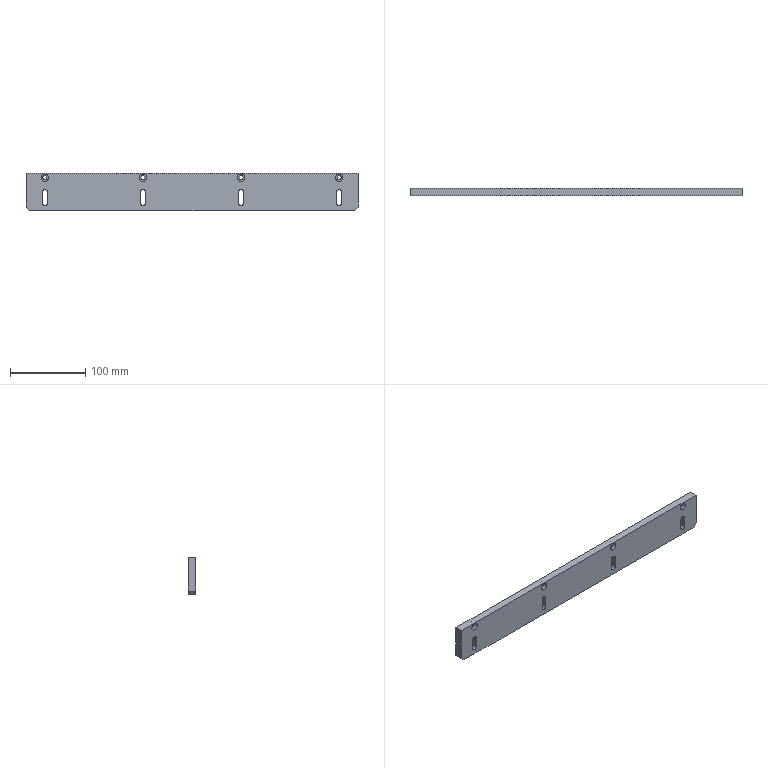Component | SolidWorks | 002MaterialPickingModuleB-1_J-019-1 | 1 solid | 48 faces | box 440 x 10 x 50 mm | volume 212389 mm3 | cylinder 28 | plane 20 | commonest cylinder face diameters 6.5 x12 10 x8 5.5 x8 | material 45
build123d program:
from build123d import *

# Parameters (mm, degrees)
SKETCH1_W                                       = 440
SKETCH1_H                                       = 50
BOSS_EXTRUDE1_DEPTH                             = 10
CHAMFER1_SIZE                                   = 5
M5_HEX_SOCKET_HEAD_CAP_SCREW_CBORE1_D           = 5.5
M5_HEX_SOCKET_HEAD_CAP_SCREW_CBORE1_CBORE_D     = 10
M5_HEX_SOCKET_HEAD_CAP_SCREW_CBORE1_CBORE_DEPTH = 5.4
CUT_EXTRUDE1_DEPTH                              = 222.642


with BuildPart() as part:
    # Sketch1 → Boss-Extrude1 (new body)
    with BuildSketch(Plane(origin=(0, 0, 0), x_dir=(1, 0, 0), z_dir=(0, 1, 0))):
        Rectangle(SKETCH1_W, SKETCH1_H)
    extrude(amount=BOSS_EXTRUDE1_DEPTH)

    # Chamfer1
    chamfer1_edges = [part.edges().sort_by_distance(p)[0] for p in [
        (-220, 5, -25),
        (220, 5, -25),
    ]]
    chamfer(chamfer1_edges, length=CHAMFER1_SIZE)

    # M5 Hex Socket Head Cap Screw CBORE1 (through all)
    with Locations(Plane(origin=(0, 0, 0), x_dir=(-1, 0, 0), z_dir=(0, -1, 0))):
        with Locations((-195, -19), (-65, -19), (65, -19), (195, -19)):
            CounterBoreHole(M5_HEX_SOCKET_HEAD_CAP_SCREW_CBORE1_D / 2, M5_HEX_SOCKET_HEAD_CAP_SCREW_CBORE1_CBORE_D / 2, M5_HEX_SOCKET_HEAD_CAP_SCREW_CBORE1_CBORE_DEPTH)

    # Sketch4 → Cut-Extrude1 (cut, through all)
    with BuildSketch(Plane(origin=(0, 10, 0), x_dir=(1, 0, 0), z_dir=(0, 1, 0))):
        with BuildLine():
            Line((-198.25, 0), (-198.25, 15))
            ThreePointArc((-198.25, 15), (-195, 18.25), (-191.75, 15))
            Line((-191.75, 15), (-191.75, 0))
            ThreePointArc((-191.75, 0), (-195, -3.25), (-198.25, 0))
        make_face()
        with BuildLine():
            Line((-68.25, 0), (-68.25, 15))
            ThreePointArc((-68.25, 15), (-65, 18.25), (-61.75, 15))
            Line((-61.75, 15), (-61.75, 0))
            ThreePointArc((-61.75, 0), (-65, -3.25), (-68.25, 0))
        make_face()
        with BuildLine():
            Line((61.75, 0), (61.75, 15))
            ThreePointArc((61.75, 15), (65, 18.25), (68.25, 15))
            Line((68.25, 15), (68.25, 0))
            ThreePointArc((68.25, 0), (65, -3.25), (61.75, 0))
        make_face()
        with BuildLine():
            Line((191.75, 0), (191.75, 15))
            ThreePointArc((191.75, 15), (195, 18.25), (198.25, 15))
            Line((198.25, 15), (198.25, 0))
            ThreePointArc((198.25, 0), (195, -3.25), (191.75, 0))
        make_face()
    extrude(amount=-CUT_EXTRUDE1_DEPTH, mode=Mode.SUBTRACT)


solid = part.part

# Placed as in the assembly
solid = solid.moved(Location((220.325, 21.019, 100.231), (0, 0, 0)))